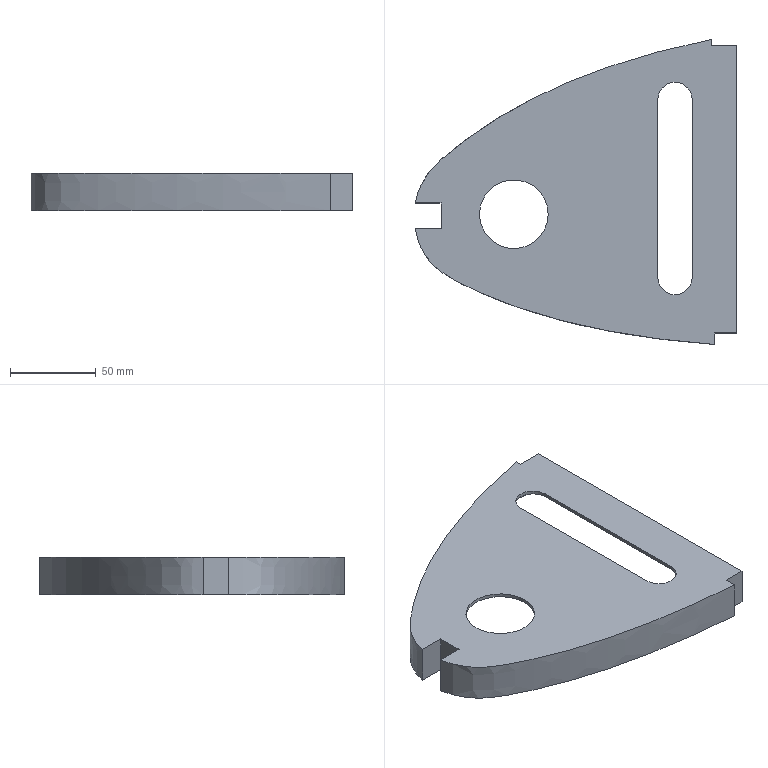Component | NX | FRONT_RIB | 1 solid | 28 faces | volume 67262 mm3 | plane 21 | cylinder 3 | other 2 | spline 2 | commonest cylinder face diameters 20 x2 40 x1